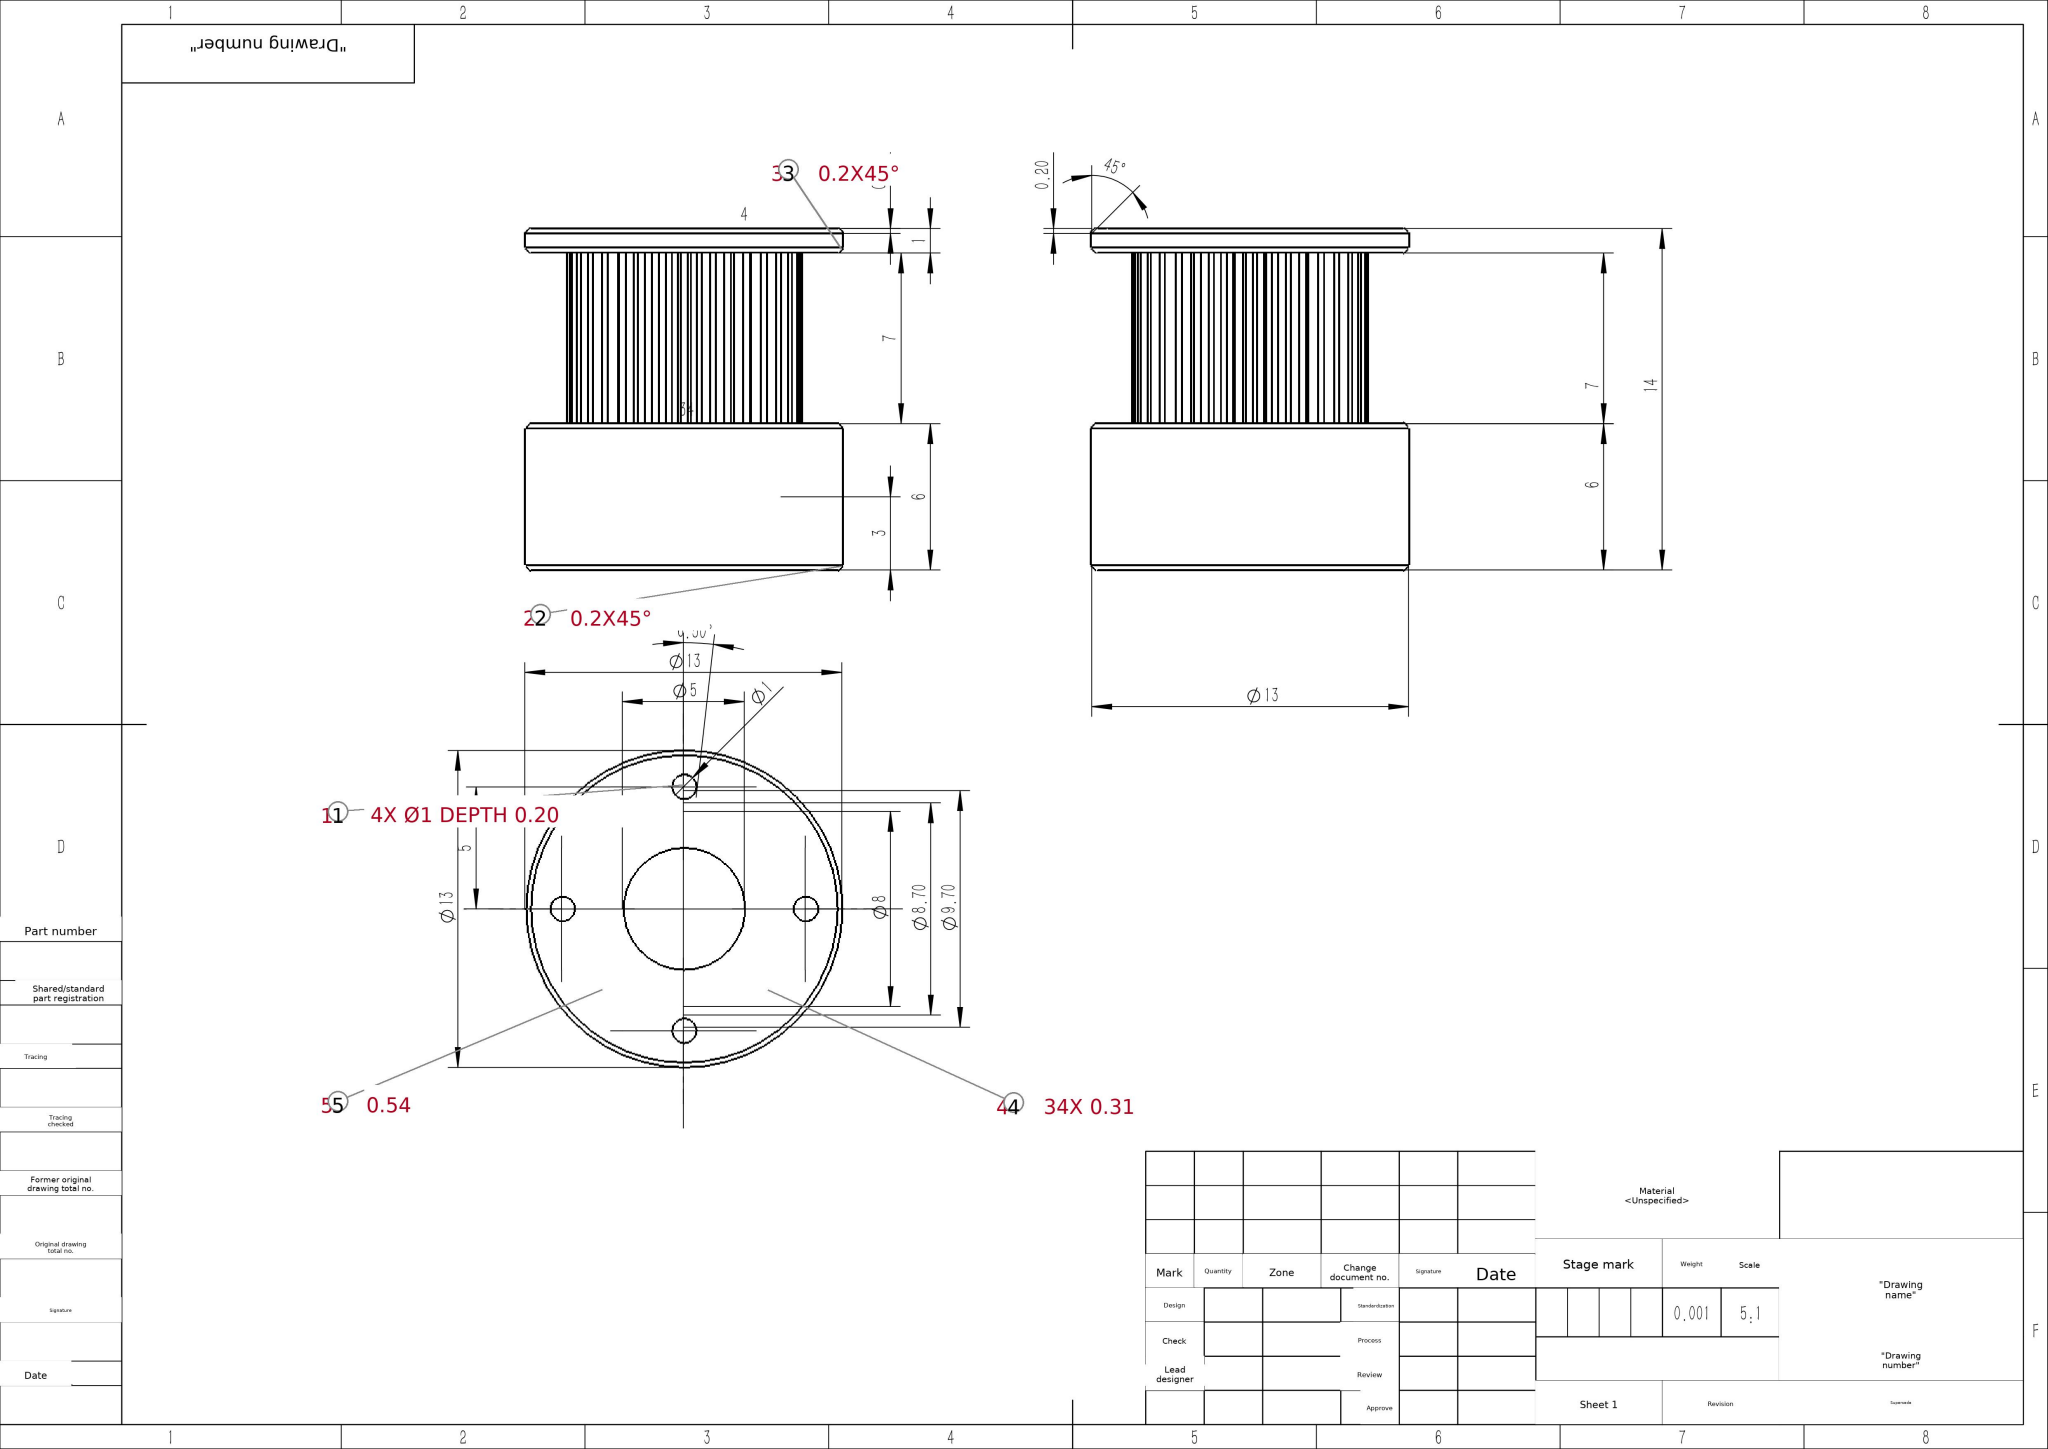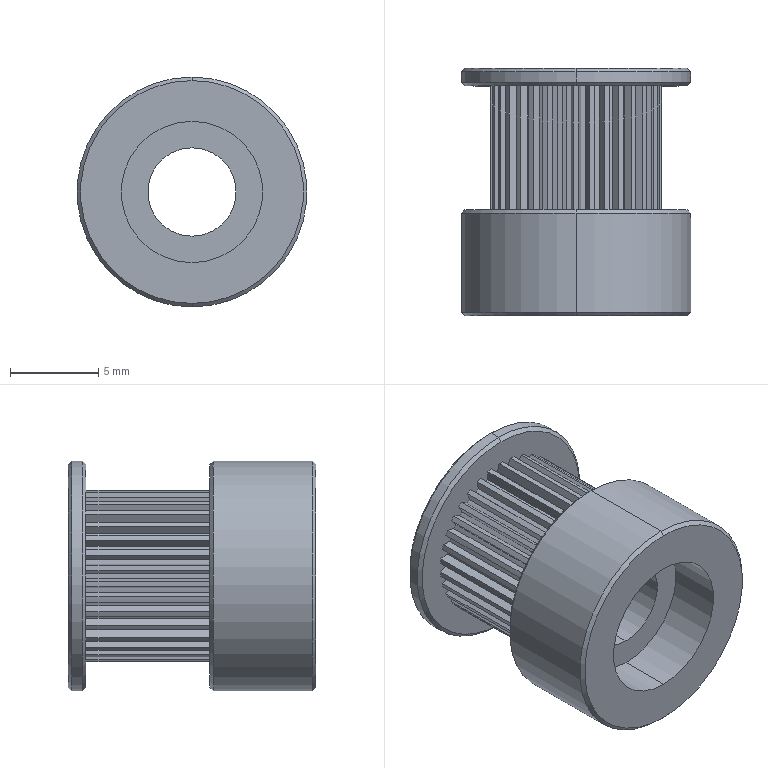Part | SolidWorks | mm | 1 solid | 170 faces | box 13 x 14 x 13 mm | volume 1025 mm3 | cylinder 85 | plane 77 | cone 8 | commonest cylinder face diameters 9.7 x35 8.7 x34 1 x8 13 x4 8 x2 5 x2
build123d program:
from build123d import *

# Parameters (mm, degrees)
SKETCH1_R           = 6.5
SKETCH1_R_2         = 2.5
BOSS_EXTRUDE1_DEPTH = 6
SKETCH4_R           = 2.5
BOSS_EXTRUDE4_DEPTH = 7
SKETCH5_R           = 6.5
SKETCH5_R_2         = 2.5
BOSS_EXTRUDE5_DEPTH = 1
CHAMFER1_SIZE       = 0.2
SKETCH6_R           = 4
CUT_EXTRUDE1_DEPTH  = 3
SKETCH7_R           = 0.5
CUT_EXTRUDE2_DEPTH  = 0.2


with BuildPart() as part:
    # Sketch1 → Boss-Extrude1 (new body)
    with BuildSketch(Plane(origin=(0, 0, 0), x_dir=(1, 0, 0), z_dir=(0, 1, 0))):
        with Locations(Location((0, 0, 0), (0, 0, 270))):
            Circle(SKETCH1_R)
        with Locations(Location((0, 0, 0), (0, 0, 270))):
            Circle(SKETCH1_R_2, mode=Mode.SUBTRACT)
    extrude(amount=BOSS_EXTRUDE1_DEPTH)

    # Sketch4 → Boss-Extrude4 (add)
    with BuildSketch(Plane(origin=(0, 6, 0), x_dir=(1, 0, 0), z_dir=(0, 1, 0))):
        with BuildLine():
            Line((-0.2692, 4.342), (-0.1534, 4.848))
            ThreePointArc((-0.1534, 4.848), (0, 4.85), (0.1534, 4.848))
            Line((0.1534, 4.848), (0.2692, 4.342))
            ThreePointArc((0.2692, 4.342), (0.4014, 4.331), (0.5332, 4.317))
            Line((0.5332, 4.317), (0.7399, 4.793))
            ThreePointArc((0.7399, 4.793), (0.8912, 4.767), (1.042, 4.737))
            Line((1.042, 4.737), (1.062, 4.218))
            ThreePointArc((1.062, 4.218), (1.19, 4.184), (1.317, 4.146))
            Line((1.317, 4.146), (1.608, 4.576))
            ThreePointArc((1.608, 4.576), (1.752, 4.522), (1.894, 4.465))
            Line((1.894, 4.465), (1.819, 3.951))
            ThreePointArc((1.819, 3.951), (1.939, 3.894), (2.057, 3.833))
            Line((2.057, 3.833), (2.421, 4.202))
            ThreePointArc((2.421, 4.202), (2.553, 4.124), (2.682, 4.041))
            Line((2.682, 4.041), (2.514, 3.55))
            ThreePointArc((2.514, 3.55), (2.621, 3.471), (2.726, 3.39))
            Line((2.726, 3.39), (3.152, 3.686))
            ThreePointArc((3.152, 3.686), (3.267, 3.584), (3.379, 3.479))
            Line((3.379, 3.479), (3.124, 3.027))
            ThreePointArc((3.124, 3.027), (3.215, 2.931), (3.303, 2.831))
            Line((3.303, 2.831), (3.776, 3.044))
            ThreePointArc((3.776, 3.044), (3.87, 2.923), (3.961, 2.799))
            Line((3.961, 2.799), (3.627, 2.402))
            ThreePointArc((3.627, 2.402), (3.698, 2.29), (3.767, 2.176))
            Line((3.767, 2.176), (4.271, 2.298))
            ThreePointArc((4.271, 2.298), (4.342, 2.162), (4.408, 2.023))
            Line((4.408, 2.023), (4.006, 1.694))
            ThreePointArc((4.006, 1.694), (4.056, 1.571), (4.102, 1.447))
            Line((4.102, 1.447), (4.621, 1.474))
            ThreePointArc((4.621, 1.474), (4.665, 1.327), (4.705, 1.179))
            Line((4.705, 1.179), (4.25, 0.9293))
            ThreePointArc((4.25, 0.9293), (4.276, 0.7993), (4.298, 0.6686))
            Line((4.298, 0.6686), (4.813, 0.6))
            ThreePointArc((4.813, 0.6), (4.829, 0.4475), (4.841, 0.2945))
            Line((4.841, 0.2945), (4.348, 0.1326))
            ThreePointArc((4.348, 0.1326), (4.35, 0), (4.348, -0.1326))
            Line((4.348, -0.1326), (4.841, -0.2945))
            ThreePointArc((4.841, -0.2945), (4.829, -0.4475), (4.813, -0.6))
            Line((4.813, -0.6), (4.298, -0.6686))
            ThreePointArc((4.298, -0.6686), (4.276, -0.7993), (4.25, -0.9293))
            Line((4.25, -0.9293), (4.705, -1.179))
            ThreePointArc((4.705, -1.179), (4.665, -1.327), (4.621, -1.474))
            Line((4.621, -1.474), (4.102, -1.447))
            ThreePointArc((4.102, -1.447), (4.056, -1.571), (4.006, -1.694))
            Line((4.006, -1.694), (4.408, -2.023))
            ThreePointArc((4.408, -2.023), (4.342, -2.162), (4.271, -2.298))
            Line((4.271, -2.298), (3.767, -2.176))
            ThreePointArc((3.767, -2.176), (3.698, -2.29), (3.627, -2.402))
            Line((3.627, -2.402), (3.961, -2.799))
            ThreePointArc((3.961, -2.799), (3.87, -2.923), (3.776, -3.044))
            Line((3.776, -3.044), (3.303, -2.831))
            ThreePointArc((3.303, -2.831), (3.215, -2.931), (3.124, -3.027))
            Line((3.124, -3.027), (3.379, -3.479))
            ThreePointArc((3.379, -3.479), (3.267, -3.584), (3.152, -3.686))
            Line((3.152, -3.686), (2.726, -3.39))
            ThreePointArc((2.726, -3.39), (2.621, -3.471), (2.514, -3.55))
            Line((2.514, -3.55), (2.682, -4.041))
            ThreePointArc((2.682, -4.041), (2.553, -4.124), (2.421, -4.202))
            Line((2.421, -4.202), (2.057, -3.833))
            ThreePointArc((2.057, -3.833), (1.939, -3.894), (1.819, -3.951))
            Line((1.819, -3.951), (1.894, -4.465))
            ThreePointArc((1.894, -4.465), (1.752, -4.522), (1.608, -4.576))
            Line((1.608, -4.576), (1.317, -4.146))
            ThreePointArc((1.317, -4.146), (1.19, -4.184), (1.062, -4.218))
            Line((1.062, -4.218), (1.042, -4.737))
            ThreePointArc((1.042, -4.737), (0.8912, -4.767), (0.7399, -4.793))
            Line((0.7399, -4.793), (0.5332, -4.317))
            ThreePointArc((0.5332, -4.317), (0.4014, -4.331), (0.2692, -4.342))
            Line((0.2692, -4.342), (0.1534, -4.848))
            ThreePointArc((0.1534, -4.848), (0, -4.85), (-0.1534, -4.848))
            Line((-0.1534, -4.848), (-0.2692, -4.342))
            ThreePointArc((-0.2692, -4.342), (-0.4014, -4.331), (-0.5332, -4.317))
            Line((-0.5332, -4.317), (-0.7399, -4.793))
            ThreePointArc((-0.7399, -4.793), (-0.8912, -4.767), (-1.042, -4.737))
            Line((-1.042, -4.737), (-1.062, -4.218))
            ThreePointArc((-1.062, -4.218), (-1.19, -4.184), (-1.317, -4.146))
            Line((-1.317, -4.146), (-1.608, -4.576))
            ThreePointArc((-1.608, -4.576), (-1.752, -4.522), (-1.894, -4.465))
            Line((-1.894, -4.465), (-1.819, -3.951))
            ThreePointArc((-1.819, -3.951), (-1.939, -3.894), (-2.057, -3.833))
            Line((-2.057, -3.833), (-2.421, -4.202))
            ThreePointArc((-2.421, -4.202), (-2.553, -4.124), (-2.682, -4.041))
            Line((-2.682, -4.041), (-2.514, -3.55))
            ThreePointArc((-2.514, -3.55), (-2.621, -3.471), (-2.726, -3.39))
            Line((-2.726, -3.39), (-3.152, -3.686))
            ThreePointArc((-3.152, -3.686), (-3.267, -3.584), (-3.379, -3.479))
            Line((-3.379, -3.479), (-3.124, -3.027))
            ThreePointArc((-3.124, -3.027), (-3.215, -2.931), (-3.303, -2.831))
            Line((-3.303, -2.831), (-3.776, -3.044))
            ThreePointArc((-3.776, -3.044), (-3.87, -2.923), (-3.961, -2.799))
            Line((-3.961, -2.799), (-3.627, -2.402))
            ThreePointArc((-3.627, -2.402), (-3.698, -2.29), (-3.767, -2.176))
            Line((-3.767, -2.176), (-4.271, -2.298))
            ThreePointArc((-4.271, -2.298), (-4.342, -2.162), (-4.408, -2.023))
            Line((-4.408, -2.023), (-4.006, -1.694))
            ThreePointArc((-4.006, -1.694), (-4.056, -1.571), (-4.102, -1.447))
            Line((-4.102, -1.447), (-4.621, -1.474))
            ThreePointArc((-4.621, -1.474), (-4.665, -1.327), (-4.705, -1.179))
            Line((-4.705, -1.179), (-4.25, -0.9293))
            ThreePointArc((-4.25, -0.9293), (-4.276, -0.7993), (-4.298, -0.6686))
            Line((-4.298, -0.6686), (-4.813, -0.6))
            ThreePointArc((-4.813, -0.6), (-4.829, -0.4475), (-4.841, -0.2945))
            Line((-4.841, -0.2945), (-4.348, -0.1326))
            ThreePointArc((-4.348, -0.1326), (-4.35, 0), (-4.348, 0.1326))
            Line((-4.348, 0.1326), (-4.841, 0.2945))
            ThreePointArc((-4.841, 0.2945), (-4.829, 0.4475), (-4.813, 0.6))
            Line((-4.813, 0.6), (-4.298, 0.6686))
            ThreePointArc((-4.298, 0.6686), (-4.276, 0.7993), (-4.25, 0.9293))
            Line((-4.25, 0.9293), (-4.705, 1.179))
            ThreePointArc((-4.705, 1.179), (-4.665, 1.327), (-4.621, 1.474))
            Line((-4.621, 1.474), (-4.102, 1.447))
            ThreePointArc((-4.102, 1.447), (-4.056, 1.571), (-4.006, 1.694))
            Line((-4.006, 1.694), (-4.408, 2.023))
            ThreePointArc((-4.408, 2.023), (-4.342, 2.162), (-4.271, 2.298))
            Line((-4.271, 2.298), (-3.767, 2.176))
            ThreePointArc((-3.767, 2.176), (-3.698, 2.29), (-3.627, 2.402))
            Line((-3.627, 2.402), (-3.961, 2.799))
            ThreePointArc((-3.961, 2.799), (-3.87, 2.923), (-3.776, 3.044))
            Line((-3.776, 3.044), (-3.303, 2.831))
            ThreePointArc((-3.303, 2.831), (-3.215, 2.931), (-3.124, 3.027))
            Line((-3.124, 3.027), (-3.379, 3.479))
            ThreePointArc((-3.379, 3.479), (-3.267, 3.584), (-3.152, 3.686))
            Line((-3.152, 3.686), (-2.726, 3.39))
            ThreePointArc((-2.726, 3.39), (-2.621, 3.471), (-2.514, 3.55))
            Line((-2.514, 3.55), (-2.682, 4.041))
            ThreePointArc((-2.682, 4.041), (-2.553, 4.124), (-2.421, 4.202))
            Line((-2.421, 4.202), (-2.057, 3.833))
            ThreePointArc((-2.057, 3.833), (-1.939, 3.894), (-1.819, 3.951))
            Line((-1.819, 3.951), (-1.894, 4.465))
            ThreePointArc((-1.894, 4.465), (-1.752, 4.522), (-1.608, 4.576))
            Line((-1.608, 4.576), (-1.317, 4.146))
            ThreePointArc((-1.317, 4.146), (-1.19, 4.184), (-1.062, 4.218))
            Line((-1.062, 4.218), (-1.042, 4.737))
            ThreePointArc((-1.042, 4.737), (-0.8912, 4.767), (-0.7399, 4.793))
            Line((-0.7399, 4.793), (-0.5332, 4.317))
            ThreePointArc((-0.5332, 4.317), (-0.4014, 4.331), (-0.2692, 4.342))
        make_face()
        with Locations(Location((0, 0, 0), (0, 0, 270))):
            Circle(SKETCH4_R, mode=Mode.SUBTRACT)
    extrude(amount=BOSS_EXTRUDE4_DEPTH)

    # Sketch5 → Boss-Extrude5 (add)
    with BuildSketch(Plane(origin=(0, 13, 0), x_dir=(1, 0, 0), z_dir=(0, 1, 0))):
        with Locations(Location((0, 0, 0), (0, 0, 270))):
            Circle(SKETCH5_R)
        with Locations(Location((0, 0, 0), (0, 0, 270))):
            Circle(SKETCH5_R_2, mode=Mode.SUBTRACT)
    extrude(amount=BOSS_EXTRUDE5_DEPTH)

    # Chamfer1
    chamfer1_edges = [part.edges().sort_by_distance(p)[0] for p in [
        (0, 0, -6.5),
        (0, 14, -6.5),
        (0, 13, -6.5),
        (0, 6, -6.5),
    ]]
    chamfer(chamfer1_edges, length=CHAMFER1_SIZE)

    # Sketch6 → Cut-Extrude1 (cut)
    with BuildSketch(Plane.XZ):
        with Locations(Location((0, 0, 0), (0, 0, 270))):
            Circle(SKETCH6_R)
    extrude(amount=-CUT_EXTRUDE1_DEPTH, mode=Mode.SUBTRACT)

    # Sketch7 → Cut-Extrude2 (cut)
    with BuildSketch(Plane(origin=(0, 14, 0), x_dir=(1, 0, 0), z_dir=(0, 1, 0))):
        with Locations(Location((0, 5, 0), (0, 0, 270))):
            Circle(SKETCH7_R)
        with Locations(Location((5, 0, 0), (0, 0, 270))):
            Circle(SKETCH7_R)
        with Locations(Location((0, -5, 0), (0, 0, 270))):
            Circle(SKETCH7_R)
        with Locations(Location((-5, 0, 0), (0, 0, 270))):
            Circle(SKETCH7_R)
    extrude(amount=-CUT_EXTRUDE2_DEPTH, mode=Mode.SUBTRACT)


solid = part.part